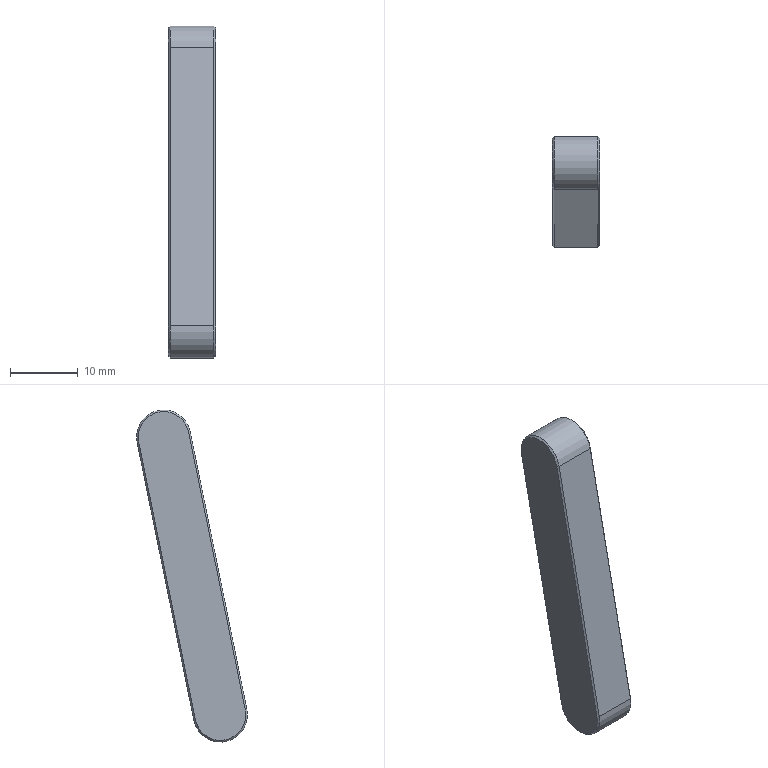Component | SolidWorks | Key_8-50-1 | 1 solid | 14 faces | box 7 x 16.4 x 49.15 mm | volume 2697 mm3 | plane 8 | cone 4 | cylinder 2 | commonest cylinder face diameters 8 x2
STEP:
#1=COLOUR_RGB('',0.7922,0.8196,0.9333);
#2=FILL_AREA_STYLE_COLOUR('',#1);
#3=FILL_AREA_STYLE('',(#2));
#4=SURFACE_STYLE_FILL_AREA(#3);
#5=SURFACE_SIDE_STYLE('',(#4));
#6=SURFACE_STYLE_USAGE(.BOTH.,#5);
#7=PRESENTATION_STYLE_ASSIGNMENT((#6));
#8=CARTESIAN_POINT('',(0.3445,6.797,-0.1417));
#9=VERTEX_POINT('',#8);
#10=CARTESIAN_POINT('',(0.6004,6.797,-0.1417));
#11=VERTEX_POINT('',#10);
#12=CARTESIAN_POINT('',(0.3346,6.797,-0.1417));
#13=DIRECTION('',(1.,-0.,-0.));
#14=VECTOR('',#13,39.37);
#15=LINE('',#12,#14);
#16=EDGE_CURVE('',#9,#11,#15,.T.);
#17=ORIENTED_EDGE('',*,*,#16,.T.);
#18=CARTESIAN_POINT('',(0.6004,6.466,-1.762));
#19=VERTEX_POINT('',#18);
#20=CARTESIAN_POINT('',(0.6004,6.466,-1.762));
#21=DIRECTION('',(-0.,-0.2,-0.9798));
#22=VECTOR('',#21,39.37);
#23=LINE('',#20,#22);
#24=EDGE_CURVE('',#11,#19,#23,.T.);
#25=ORIENTED_EDGE('',*,*,#24,.T.);
#26=CARTESIAN_POINT('',(0.3445,6.466,-1.762));
#27=VERTEX_POINT('',#26);
#28=CARTESIAN_POINT('',(0.3346,6.466,-1.762));
#29=DIRECTION('',(1.,-0.,-0.));
#30=VECTOR('',#29,39.37);
#31=LINE('',#28,#30);
#32=EDGE_CURVE('',#27,#19,#31,.T.);
#33=ORIENTED_EDGE('',*,*,#32,.F.);
#34=CARTESIAN_POINT('',(0.3445,6.829,0.0126));
#35=DIRECTION('',(0.,0.2,0.9798));
#36=VECTOR('',#35,39.37);
#37=LINE('',#34,#36);
#38=EDGE_CURVE('',#27,#9,#37,.T.);
#39=ORIENTED_EDGE('',*,*,#38,.T.);
#40=EDGE_LOOP('',(#17,#25,#33,#39));
#41=FACE_OUTER_BOUND('',#40,.T.);
#42=CARTESIAN_POINT('',(0.3346,6.829,0.0126));
#43=DIRECTION('',(-0.,-0.9798,0.2));
#44=DIRECTION('',(0.,0.2,0.9798));
#45=AXIS2_PLACEMENT_3D('',#42,#43,#44);
#46=PLANE('',#45);
#47=ADVANCED_FACE('',(#41),#46,.F.);
#48=CARTESIAN_POINT('',(0.3445,6.158,-1.699));
#49=VERTEX_POINT('',#48);
#50=CARTESIAN_POINT('',(0.6004,6.158,-1.699));
#51=VERTEX_POINT('',#50);
#52=CARTESIAN_POINT('',(0.3346,6.158,-1.699));
#53=DIRECTION('',(1.,-0.,-0.));
#54=VECTOR('',#53,39.37);
#55=LINE('',#52,#54);
#56=EDGE_CURVE('',#49,#51,#55,.T.);
#57=ORIENTED_EDGE('',*,*,#56,.T.);
#58=CARTESIAN_POINT('',(0.6004,6.489,-0.07872));
#59=VERTEX_POINT('',#58);
#60=CARTESIAN_POINT('',(0.6004,6.489,-0.07872));
#61=DIRECTION('',(0.,0.2,0.9798));
#62=VECTOR('',#61,39.37);
#63=LINE('',#60,#62);
#64=EDGE_CURVE('',#51,#59,#63,.T.);
#65=ORIENTED_EDGE('',*,*,#64,.T.);
#66=CARTESIAN_POINT('',(0.3445,6.489,-0.07872));
#67=VERTEX_POINT('',#66);
#68=CARTESIAN_POINT('',(0.3346,6.489,-0.07872));
#69=DIRECTION('',(1.,-0.,-0.));
#70=VECTOR('',#69,39.37);
#71=LINE('',#68,#70);
#72=EDGE_CURVE('',#67,#59,#71,.T.);
#73=ORIENTED_EDGE('',*,*,#72,.F.);
#74=CARTESIAN_POINT('',(0.3445,6.52,0.07558));
#75=DIRECTION('',(-0.,-0.2,-0.9798));
#76=VECTOR('',#75,39.37);
#77=LINE('',#74,#76);
#78=EDGE_CURVE('',#67,#49,#77,.T.);
#79=ORIENTED_EDGE('',*,*,#78,.T.);
#80=EDGE_LOOP('',(#57,#65,#73,#79));
#81=FACE_OUTER_BOUND('',#80,.T.);
#82=CARTESIAN_POINT('',(0.3346,6.52,0.07558));
#83=DIRECTION('',(0.,0.9798,-0.2));
#84=DIRECTION('',(-0.,-0.2,-0.9798));
#85=AXIS2_PLACEMENT_3D('',#82,#83,#84);
#86=PLANE('',#85);
#87=ADVANCED_FACE('',(#81),#86,.F.);
#88=CARTESIAN_POINT('',(0.3346,6.457,-1.76));
#89=VERTEX_POINT('',#88);
#90=CARTESIAN_POINT('',(0.3346,6.168,-1.701));
#91=VERTEX_POINT('',#90);
#92=CARTESIAN_POINT('',(0.3346,6.312,-1.73));
#93=DIRECTION('',(-1.,0.,0.));
#94=DIRECTION('',(0.,-0.9798,0.2));
#95=AXIS2_PLACEMENT_3D('',#92,#93,#94);
#96=CIRCLE('',#95,0.1476);
#97=EDGE_CURVE('',#89,#91,#96,.T.);
#98=ORIENTED_EDGE('',*,*,#97,.T.);
#99=CARTESIAN_POINT('',(0.3346,6.498,-0.08069));
#100=VERTEX_POINT('',#99);
#101=CARTESIAN_POINT('',(0.3346,6.53,0.07361));
#102=DIRECTION('',(0.,0.2,0.9798));
#103=VECTOR('',#102,39.37);
#104=LINE('',#101,#103);
#105=EDGE_CURVE('',#91,#100,#104,.T.);
#106=ORIENTED_EDGE('',*,*,#105,.T.);
#107=CARTESIAN_POINT('',(0.3346,6.787,-0.1397));
#108=VERTEX_POINT('',#107);
#109=CARTESIAN_POINT('',(0.3346,6.643,-0.1102));
#110=DIRECTION('',(-1.,0.,0.));
#111=DIRECTION('',(0.,-0.9798,0.2));
#112=AXIS2_PLACEMENT_3D('',#109,#110,#111);
#113=CIRCLE('',#112,0.1476);
#114=EDGE_CURVE('',#100,#108,#113,.T.);
#115=ORIENTED_EDGE('',*,*,#114,.T.);
#116=CARTESIAN_POINT('',(0.3346,6.819,0.01456));
#117=DIRECTION('',(-0.,-0.2,-0.9798));
#118=VECTOR('',#117,39.37);
#119=LINE('',#116,#118);
#120=EDGE_CURVE('',#108,#89,#119,.T.);
#121=ORIENTED_EDGE('',*,*,#120,.T.);
#122=EDGE_LOOP('',(#98,#106,#115,#121));
#123=FACE_OUTER_BOUND('',#122,.T.);
#124=CARTESIAN_POINT('',(0.3346,6.52,0.07558));
#125=DIRECTION('',(1.,-0.,-0.));
#126=DIRECTION('',(-0.,-0.9798,0.2));
#127=AXIS2_PLACEMENT_3D('',#124,#125,#126);
#128=PLANE('',#127);
#129=ADVANCED_FACE('',(#123),#128,.F.);
#130=CARTESIAN_POINT('',(0.6102,6.457,-1.76));
#131=VERTEX_POINT('',#130);
#132=CARTESIAN_POINT('',(0.6102,6.787,-0.1397));
#133=VERTEX_POINT('',#132);
#134=CARTESIAN_POINT('',(0.6102,6.787,-0.1397));
#135=DIRECTION('',(0.,0.2,0.9798));
#136=VECTOR('',#135,39.37);
#137=LINE('',#134,#136);
#138=EDGE_CURVE('',#131,#133,#137,.T.);
#139=ORIENTED_EDGE('',*,*,#138,.T.);
#140=CARTESIAN_POINT('',(0.6102,6.498,-0.08069));
#141=VERTEX_POINT('',#140);
#142=CARTESIAN_POINT('',(0.6102,6.643,-0.1102));
#143=DIRECTION('',(1.,-0.,-0.));
#144=DIRECTION('',(0.,-0.9798,0.2));
#145=AXIS2_PLACEMENT_3D('',#142,#143,#144);
#146=CIRCLE('',#145,0.1476);
#147=EDGE_CURVE('',#133,#141,#146,.T.);
#148=ORIENTED_EDGE('',*,*,#147,.T.);
#149=CARTESIAN_POINT('',(0.6102,6.168,-1.701));
#150=VERTEX_POINT('',#149);
#151=CARTESIAN_POINT('',(0.6102,6.168,-1.701));
#152=DIRECTION('',(-0.,-0.2,-0.9798));
#153=VECTOR('',#152,39.37);
#154=LINE('',#151,#153);
#155=EDGE_CURVE('',#141,#150,#154,.T.);
#156=ORIENTED_EDGE('',*,*,#155,.T.);
#157=CARTESIAN_POINT('',(0.6102,6.312,-1.73));
#158=DIRECTION('',(1.,-0.,-0.));
#159=DIRECTION('',(0.,-0.9798,0.2));
#160=AXIS2_PLACEMENT_3D('',#157,#158,#159);
#161=CIRCLE('',#160,0.1476);
#162=EDGE_CURVE('',#150,#131,#161,.T.);
#163=ORIENTED_EDGE('',*,*,#162,.T.);
#164=EDGE_LOOP('',(#139,#148,#156,#163));
#165=FACE_OUTER_BOUND('',#164,.T.);
#166=CARTESIAN_POINT('',(0.6102,6.52,0.07558));
#167=DIRECTION('',(1.,-0.,-0.));
#168=DIRECTION('',(-0.,-0.9798,0.2));
#169=AXIS2_PLACEMENT_3D('',#166,#167,#168);
#170=PLANE('',#169);
#171=ADVANCED_FACE('',(#165),#170,.T.);
#172=ORIENTED_EDGE('',*,*,#32,.T.);
#173=CARTESIAN_POINT('',(0.6004,6.312,-1.73));
#174=DIRECTION('',(-1.,0.,0.));
#175=DIRECTION('',(0.,-0.9798,0.2));
#176=AXIS2_PLACEMENT_3D('',#173,#174,#175);
#177=CIRCLE('',#176,0.1575);
#178=EDGE_CURVE('',#19,#51,#177,.T.);
#179=ORIENTED_EDGE('',*,*,#178,.T.);
#180=ORIENTED_EDGE('',*,*,#56,.F.);
#181=CARTESIAN_POINT('',(0.3445,6.312,-1.73));
#182=DIRECTION('',(1.,-0.,-0.));
#183=DIRECTION('',(0.,-0.9798,0.2));
#184=AXIS2_PLACEMENT_3D('',#181,#182,#183);
#185=CIRCLE('',#184,0.1575);
#186=EDGE_CURVE('',#49,#27,#185,.T.);
#187=ORIENTED_EDGE('',*,*,#186,.T.);
#188=EDGE_LOOP('',(#172,#179,#180,#187));
#189=FACE_OUTER_BOUND('',#188,.T.);
#190=CARTESIAN_POINT('',(0.3346,6.312,-1.73));
#191=DIRECTION('',(1.,-0.,-0.));
#192=DIRECTION('',(0.,-0.9798,0.2));
#193=AXIS2_PLACEMENT_3D('',#190,#191,#192);
#194=CYLINDRICAL_SURFACE('',#193,0.1575);
#195=ADVANCED_FACE('',(#189),#194,.T.);
#196=ORIENTED_EDGE('',*,*,#72,.T.);
#197=CARTESIAN_POINT('',(0.6004,6.643,-0.1102));
#198=DIRECTION('',(-1.,0.,0.));
#199=DIRECTION('',(0.,-0.9798,0.2));
#200=AXIS2_PLACEMENT_3D('',#197,#198,#199);
#201=CIRCLE('',#200,0.1575);
#202=EDGE_CURVE('',#59,#11,#201,.T.);
#203=ORIENTED_EDGE('',*,*,#202,.T.);
#204=ORIENTED_EDGE('',*,*,#16,.F.);
#205=CARTESIAN_POINT('',(0.3445,6.643,-0.1102));
#206=DIRECTION('',(1.,-0.,-0.));
#207=DIRECTION('',(0.,-0.9798,0.2));
#208=AXIS2_PLACEMENT_3D('',#205,#206,#207);
#209=CIRCLE('',#208,0.1575);
#210=EDGE_CURVE('',#9,#67,#209,.T.);
#211=ORIENTED_EDGE('',*,*,#210,.T.);
#212=EDGE_LOOP('',(#196,#203,#204,#211));
#213=FACE_OUTER_BOUND('',#212,.T.);
#214=CARTESIAN_POINT('',(0.3346,6.643,-0.1102));
#215=DIRECTION('',(1.,-0.,-0.));
#216=DIRECTION('',(0.,-0.9798,0.2));
#217=AXIS2_PLACEMENT_3D('',#214,#215,#216);
#218=CYLINDRICAL_SURFACE('',#217,0.1575);
#219=ADVANCED_FACE('',(#213),#218,.T.);
#220=CARTESIAN_POINT('',(0.6102,6.457,-1.76));
#221=DIRECTION('',(-0.7071,0.6928,-0.1414));
#222=VECTOR('',#221,39.37);
#223=LINE('',#220,#222);
#224=EDGE_CURVE('',#131,#19,#223,.T.);
#225=ORIENTED_EDGE('',*,*,#224,.F.);
#226=ORIENTED_EDGE('',*,*,#162,.F.);
#227=CARTESIAN_POINT('',(0.6004,6.158,-1.699));
#228=DIRECTION('',(0.7071,0.6928,-0.1414));
#229=VECTOR('',#228,39.37);
#230=LINE('',#227,#229);
#231=EDGE_CURVE('',#51,#150,#230,.T.);
#232=ORIENTED_EDGE('',*,*,#231,.F.);
#233=ORIENTED_EDGE('',*,*,#178,.F.);
#234=EDGE_LOOP('',(#225,#226,#232,#233));
#235=FACE_OUTER_BOUND('',#234,.T.);
#236=CARTESIAN_POINT('',(0.6004,6.312,-1.73));
#237=DIRECTION('',(-1.,0.,0.));
#238=DIRECTION('',(0.,0.9798,-0.2));
#239=AXIS2_PLACEMENT_3D('',#236,#237,#238);
#240=CONICAL_SURFACE('',#239,0.1575,0.7854);
#241=ADVANCED_FACE('',(#235),#240,.T.);
#242=ORIENTED_EDGE('',*,*,#231,.T.);
#243=ORIENTED_EDGE('',*,*,#155,.F.);
#244=CARTESIAN_POINT('',(0.6004,6.489,-0.07872));
#245=DIRECTION('',(0.7071,0.6928,-0.1414));
#246=VECTOR('',#245,39.37);
#247=LINE('',#244,#246);
#248=EDGE_CURVE('',#59,#141,#247,.T.);
#249=ORIENTED_EDGE('',*,*,#248,.F.);
#250=ORIENTED_EDGE('',*,*,#64,.F.);
#251=EDGE_LOOP('',(#242,#243,#249,#250));
#252=FACE_OUTER_BOUND('',#251,.T.);
#253=CARTESIAN_POINT('',(0.6004,6.52,0.07558));
#254=DIRECTION('',(0.7071,-0.6928,0.1414));
#255=DIRECTION('',(-0.7071,-0.6928,0.1414));
#256=AXIS2_PLACEMENT_3D('',#253,#254,#255);
#257=PLANE('',#256);
#258=ADVANCED_FACE('',(#252),#257,.T.);
#259=ORIENTED_EDGE('',*,*,#224,.T.);
#260=ORIENTED_EDGE('',*,*,#24,.F.);
#261=CARTESIAN_POINT('',(0.6102,6.787,-0.1397));
#262=DIRECTION('',(-0.7071,0.6928,-0.1414));
#263=VECTOR('',#262,39.37);
#264=LINE('',#261,#263);
#265=EDGE_CURVE('',#133,#11,#264,.T.);
#266=ORIENTED_EDGE('',*,*,#265,.F.);
#267=ORIENTED_EDGE('',*,*,#138,.F.);
#268=EDGE_LOOP('',(#259,#260,#266,#267));
#269=FACE_OUTER_BOUND('',#268,.T.);
#270=CARTESIAN_POINT('',(0.6004,6.829,0.0126));
#271=DIRECTION('',(0.7071,0.6928,-0.1414));
#272=DIRECTION('',(0.7071,-0.6928,0.1414));
#273=AXIS2_PLACEMENT_3D('',#270,#271,#272);
#274=PLANE('',#273);
#275=ADVANCED_FACE('',(#269),#274,.T.);
#276=ORIENTED_EDGE('',*,*,#248,.T.);
#277=ORIENTED_EDGE('',*,*,#147,.F.);
#278=ORIENTED_EDGE('',*,*,#265,.T.);
#279=ORIENTED_EDGE('',*,*,#202,.F.);
#280=EDGE_LOOP('',(#276,#277,#278,#279));
#281=FACE_OUTER_BOUND('',#280,.T.);
#282=CARTESIAN_POINT('',(0.6004,6.643,-0.1102));
#283=DIRECTION('',(-1.,0.,0.));
#284=DIRECTION('',(0.,0.9798,-0.2));
#285=AXIS2_PLACEMENT_3D('',#282,#283,#284);
#286=CONICAL_SURFACE('',#285,0.1575,0.7854);
#287=ADVANCED_FACE('',(#281),#286,.T.);
#288=CARTESIAN_POINT('',(0.3445,6.797,-0.1417));
#289=DIRECTION('',(-0.7071,-0.6928,0.1414));
#290=VECTOR('',#289,39.37);
#291=LINE('',#288,#290);
#292=EDGE_CURVE('',#9,#108,#291,.T.);
#293=ORIENTED_EDGE('',*,*,#292,.F.);
#294=ORIENTED_EDGE('',*,*,#38,.F.);
#295=CARTESIAN_POINT('',(0.3346,6.457,-1.76));
#296=DIRECTION('',(0.7071,0.6928,-0.1414));
#297=VECTOR('',#296,39.37);
#298=LINE('',#295,#297);
#299=EDGE_CURVE('',#89,#27,#298,.T.);
#300=ORIENTED_EDGE('',*,*,#299,.F.);
#301=ORIENTED_EDGE('',*,*,#120,.F.);
#302=EDGE_LOOP('',(#293,#294,#300,#301));
#303=FACE_OUTER_BOUND('',#302,.T.);
#304=CARTESIAN_POINT('',(0.3346,6.819,0.01456));
#305=DIRECTION('',(0.7071,-0.6928,0.1414));
#306=DIRECTION('',(-0.7071,-0.6928,0.1414));
#307=AXIS2_PLACEMENT_3D('',#304,#305,#306);
#308=PLANE('',#307);
#309=ADVANCED_FACE('',(#303),#308,.F.);
#310=ORIENTED_EDGE('',*,*,#299,.T.);
#311=ORIENTED_EDGE('',*,*,#186,.F.);
#312=CARTESIAN_POINT('',(0.3346,6.168,-1.701));
#313=DIRECTION('',(0.7071,-0.6928,0.1414));
#314=VECTOR('',#313,39.37);
#315=LINE('',#312,#314);
#316=EDGE_CURVE('',#91,#49,#315,.T.);
#317=ORIENTED_EDGE('',*,*,#316,.F.);
#318=ORIENTED_EDGE('',*,*,#97,.F.);
#319=EDGE_LOOP('',(#310,#311,#317,#318));
#320=FACE_OUTER_BOUND('',#319,.T.);
#321=CARTESIAN_POINT('',(0.3346,6.312,-1.73));
#322=DIRECTION('',(1.,-0.,-0.));
#323=DIRECTION('',(0.,-0.9798,0.2));
#324=AXIS2_PLACEMENT_3D('',#321,#322,#323);
#325=CONICAL_SURFACE('',#324,0.1476,0.7854);
#326=ADVANCED_FACE('',(#320),#325,.T.);
#327=ORIENTED_EDGE('',*,*,#292,.T.);
#328=ORIENTED_EDGE('',*,*,#114,.F.);
#329=CARTESIAN_POINT('',(0.3445,6.489,-0.07872));
#330=DIRECTION('',(-0.7071,0.6928,-0.1414));
#331=VECTOR('',#330,39.37);
#332=LINE('',#329,#331);
#333=EDGE_CURVE('',#67,#100,#332,.T.);
#334=ORIENTED_EDGE('',*,*,#333,.F.);
#335=ORIENTED_EDGE('',*,*,#210,.F.);
#336=EDGE_LOOP('',(#327,#328,#334,#335));
#337=FACE_OUTER_BOUND('',#336,.T.);
#338=CARTESIAN_POINT('',(0.3346,6.643,-0.1102));
#339=DIRECTION('',(1.,-0.,-0.));
#340=DIRECTION('',(0.,-0.9798,0.2));
#341=AXIS2_PLACEMENT_3D('',#338,#339,#340);
#342=CONICAL_SURFACE('',#341,0.1476,0.7854);
#343=ADVANCED_FACE('',(#337),#342,.T.);
#344=ORIENTED_EDGE('',*,*,#316,.T.);
#345=ORIENTED_EDGE('',*,*,#78,.F.);
#346=ORIENTED_EDGE('',*,*,#333,.T.);
#347=ORIENTED_EDGE('',*,*,#105,.F.);
#348=EDGE_LOOP('',(#344,#345,#346,#347));
#349=FACE_OUTER_BOUND('',#348,.T.);
#350=CARTESIAN_POINT('',(0.3346,6.53,0.07361));
#351=DIRECTION('',(0.7071,0.6928,-0.1414));
#352=DIRECTION('',(0.7071,-0.6928,0.1414));
#353=AXIS2_PLACEMENT_3D('',#350,#351,#352);
#354=PLANE('',#353);
#355=ADVANCED_FACE('',(#349),#354,.F.);
#356=CLOSED_SHELL('',(#47,#87,#129,#171,#195,#219,#241,#258,#275,#287,#309,#326,#343,#355));
#357=MANIFOLD_SOLID_BREP('',#356);
#358=STYLED_ITEM('',(#7),#357);
#359=PRESENTATION_LAYER_ASSIGNMENT('','',(#358));
#360=(LENGTH_UNIT()NAMED_UNIT(*)SI_UNIT($,.METRE.));
#361=LENGTH_MEASURE_WITH_UNIT(LENGTH_MEASURE(0.0254),#360);
#362=DIMENSIONAL_EXPONENTS(1.,0.,0.,0.,0.,0.,0.);
#363=(CONVERSION_BASED_UNIT('',#361)LENGTH_UNIT()NAMED_UNIT(#362));
#364=UNCERTAINTY_MEASURE_WITH_UNIT(LENGTH_MEASURE(0.00001),#363,'','');
#365=(NAMED_UNIT(*)PLANE_ANGLE_UNIT()SI_UNIT($,.RADIAN.));
#366=(NAMED_UNIT(*)SI_UNIT($,.STERADIAN.)SOLID_ANGLE_UNIT());
#367=(GEOMETRIC_REPRESENTATION_CONTEXT(3)GLOBAL_UNCERTAINTY_ASSIGNED_CONTEXT((#364))GLOBAL_UNIT_ASSIGNED_CONTEXT((#363,#365,#366))REPRESENTATION_CONTEXT('',''));
#368=MECHANICAL_DESIGN_GEOMETRIC_PRESENTATION_REPRESENTATION('',(#358),#367);
#369=CARTESIAN_POINT('',(0.,0.,0.));
#370=DIRECTION('',(0.,0.,1.));
#371=DIRECTION('',(1.,0.,0.));
#372=AXIS2_PLACEMENT_3D('',#369,#370,#371);
#373=(LENGTH_UNIT()NAMED_UNIT(*)SI_UNIT($,.METRE.));
#374=LENGTH_MEASURE_WITH_UNIT(LENGTH_MEASURE(0.0254),#373);
#375=DIMENSIONAL_EXPONENTS(1.,0.,0.,0.,0.,0.,0.);
#376=(CONVERSION_BASED_UNIT('',#374)LENGTH_UNIT()NAMED_UNIT(#375));
#377=UNCERTAINTY_MEASURE_WITH_UNIT(LENGTH_MEASURE(0.00001),#376,'','');
#378=(NAMED_UNIT(*)PLANE_ANGLE_UNIT()SI_UNIT($,.RADIAN.));
#379=(NAMED_UNIT(*)SI_UNIT($,.STERADIAN.)SOLID_ANGLE_UNIT());
#380=(GEOMETRIC_REPRESENTATION_CONTEXT(3)GLOBAL_UNCERTAINTY_ASSIGNED_CONTEXT((#377))GLOBAL_UNIT_ASSIGNED_CONTEXT((#376,#378,#379))REPRESENTATION_CONTEXT('',''));
#381=ADVANCED_BREP_SHAPE_REPRESENTATION('',(#357,#372),#380);